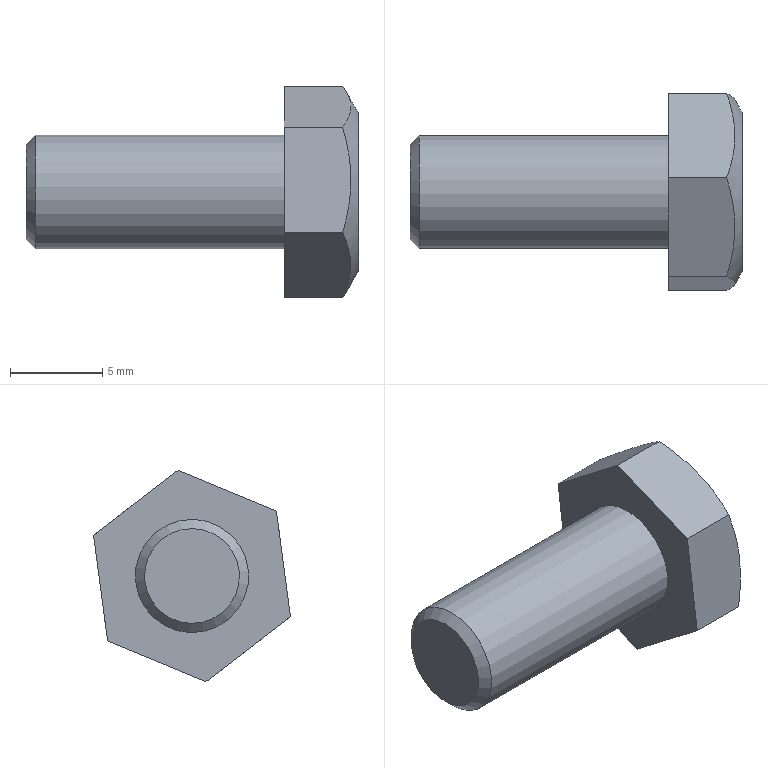Component | NX | BOLT_M6X30 | 1 solid | 12 faces | box 18 x 10.67 x 11.45 mm | volume 751 mm3 | plane 9 | cone 2 | cylinder 1 | commonest cylinder face diameters 6.144 x1
STEP:
#1=CARTESIAN_POINT('',(0.,0.,0.));
#2=DIRECTION('',(0.,0.,1.));
#3=DIRECTION('',(1.,0.,0.));
#4=AXIS2_PLACEMENT_3D('',#1,#2,#3);
#5=CARTESIAN_POINT('',(11.5,2.377,-2.015));
#6=VERTEX_POINT('',#5);
#7=CARTESIAN_POINT('',(11.5,0.,-2.997));
#8=DIRECTION('',(-1.,0.,0.));
#9=DIRECTION('',(0.,0.9242,0.3818));
#10=AXIS2_PLACEMENT_3D('',#7,#8,#9);
#11=CIRCLE('',#10,2.572);
#12=CARTESIAN_POINT('',(11.5,0.,-2.997));
#13=DIRECTION('',(-1.,0.,0.));
#14=DIRECTION('',(0.,0.9242,0.3818));
#15=AXIS2_PLACEMENT_3D('',#12,#13,#14);
#16=PLANE('',#15);
#17=CARTESIAN_POINT('',(0.,0.));
#18=DIRECTION('',(1.,0.));
#19=AXIS2_PLACEMENT_2D('',#17,#18);
#20=CIRCLE('',#19,2.572);
#21=(GEOMETRIC_REPRESENTATION_CONTEXT(2)PARAMETRIC_REPRESENTATION_CONTEXT()REPRESENTATION_CONTEXT('',''));
#22=DEFINITIONAL_REPRESENTATION('',(#20),#21);
#23=PCURVE('',#16,#22);
#24=CARTESIAN_POINT('',(12.,0.,-2.997));
#25=DIRECTION('',(1.,0.,0.));
#26=DIRECTION('',(0.,-0.9242,-0.3818));
#27=AXIS2_PLACEMENT_3D('',#24,#25,#26);
#28=CONICAL_SURFACE('',#27,3.072,0.7854);
#29=CARTESIAN_POINT('',(9.425,-0.5));
#30=DIRECTION('',(-1.,-0.));
#31=VECTOR('',#30,1.);
#32=LINE('',#29,#31);
#33=(GEOMETRIC_REPRESENTATION_CONTEXT(2)PARAMETRIC_REPRESENTATION_CONTEXT()REPRESENTATION_CONTEXT('',''));
#34=DEFINITIONAL_REPRESENTATION('',(#32),#33);
#35=PCURVE('',#28,#34);
#36=SURFACE_CURVE('',#11,(#23,#35),.PCURVE_S1.);
#37=EDGE_CURVE('',#6,#6,#36,.T.);
#38=ORIENTED_EDGE('',*,*,#37,.T.);
#39=EDGE_LOOP('',(#38));
#40=FACE_BOUND('',#39,.T.);
#41=ADVANCED_FACE('',(#40),#16,.T.);
#42=CARTESIAN_POINT('',(12.,2.839,-1.824));
#43=VERTEX_POINT('',#42);
#44=CARTESIAN_POINT('',(12.,-2.839,-4.17));
#45=VERTEX_POINT('',#44);
#46=CARTESIAN_POINT('',(12.,0.,-2.997));
#47=DIRECTION('',(1.,0.,0.));
#48=DIRECTION('',(0.,0.9242,0.3818));
#49=AXIS2_PLACEMENT_3D('',#46,#47,#48);
#50=CIRCLE('',#49,3.072);
#51=CARTESIAN_POINT('',(11.5,0.,-2.997));
#52=DIRECTION('',(1.,0.,0.));
#53=DIRECTION('',(0.,-0.9242,-0.3818));
#54=AXIS2_PLACEMENT_3D('',#51,#52,#53);
#55=CYLINDRICAL_SURFACE('',#54,3.072);
#56=CARTESIAN_POINT('',(3.142,0.5));
#57=DIRECTION('',(1.,0.));
#58=VECTOR('',#57,1.);
#59=LINE('',#56,#58);
#60=(GEOMETRIC_REPRESENTATION_CONTEXT(2)PARAMETRIC_REPRESENTATION_CONTEXT()REPRESENTATION_CONTEXT('',''));
#61=DEFINITIONAL_REPRESENTATION('',(#59),#60);
#62=PCURVE('',#55,#61);
#63=CARTESIAN_POINT('',(3.142,0.));
#64=DIRECTION('',(1.,0.));
#65=VECTOR('',#64,1.);
#66=LINE('',#63,#65);
#67=(GEOMETRIC_REPRESENTATION_CONTEXT(2)PARAMETRIC_REPRESENTATION_CONTEXT()REPRESENTATION_CONTEXT('',''));
#68=DEFINITIONAL_REPRESENTATION('',(#66),#67);
#69=PCURVE('',#28,#68);
#70=SURFACE_CURVE('',#50,(#62,#69),.PCURVE_S1.);
#71=EDGE_CURVE('',#43,#45,#70,.T.);
#72=ORIENTED_EDGE('',*,*,#71,.T.);
#73=CARTESIAN_POINT('',(25.5,-2.839,-4.17));
#74=VERTEX_POINT('',#73);
#75=CARTESIAN_POINT('',(12.,-2.839,-4.17));
#76=CARTESIAN_POINT('',(25.5,-2.839,-4.17));
#77=B_SPLINE_CURVE_WITH_KNOTS('',1,(#75,#76),.UNSPECIFIED.,.F.,.F.,(2,2),(0.5,14.),.PIECEWISE_BEZIER_KNOTS.);
#78=CARTESIAN_POINT('',(6.283,0.));
#79=DIRECTION('',(0.,1.));
#80=VECTOR('',#79,1.);
#81=LINE('',#78,#80);
#82=(GEOMETRIC_REPRESENTATION_CONTEXT(2)PARAMETRIC_REPRESENTATION_CONTEXT()REPRESENTATION_CONTEXT('',''));
#83=DEFINITIONAL_REPRESENTATION('',(#81),#82);
#84=PCURVE('',#55,#83);
#85=CARTESIAN_POINT('',(0.,0.));
#86=DIRECTION('',(0.,1.));
#87=VECTOR('',#86,1.);
#88=LINE('',#85,#87);
#89=(GEOMETRIC_REPRESENTATION_CONTEXT(2)PARAMETRIC_REPRESENTATION_CONTEXT()REPRESENTATION_CONTEXT('',''));
#90=DEFINITIONAL_REPRESENTATION('',(#88),#89);
#91=PCURVE('',#55,#90);
#92=SEAM_CURVE('',#77,(#84,#91),.PCURVE_S1.);
#93=EDGE_CURVE('',#45,#74,#92,.T.);
#94=ORIENTED_EDGE('',*,*,#93,.T.);
#95=CARTESIAN_POINT('',(25.5,0.,-2.997));
#96=DIRECTION('',(-1.,0.,0.));
#97=DIRECTION('',(0.,-0.9242,-0.3818));
#98=AXIS2_PLACEMENT_3D('',#95,#96,#97);
#99=CIRCLE('',#98,3.072);
#100=CARTESIAN_POINT('',(6.283,14.));
#101=DIRECTION('',(-1.,0.));
#102=VECTOR('',#101,1.);
#103=LINE('',#100,#102);
#104=(GEOMETRIC_REPRESENTATION_CONTEXT(2)PARAMETRIC_REPRESENTATION_CONTEXT()REPRESENTATION_CONTEXT('',''));
#105=DEFINITIONAL_REPRESENTATION('',(#103),#104);
#106=PCURVE('',#55,#105);
#107=CARTESIAN_POINT('',(25.5,0.,-2.997));
#108=DIRECTION('',(-1.,0.,0.));
#109=DIRECTION('',(0.,0.9242,0.3818));
#110=AXIS2_PLACEMENT_3D('',#107,#108,#109);
#111=PLANE('',#110);
#112=CARTESIAN_POINT('',(0.,0.));
#113=DIRECTION('',(-1.,0.));
#114=AXIS2_PLACEMENT_2D('',#112,#113);
#115=CIRCLE('',#114,3.072);
#116=(GEOMETRIC_REPRESENTATION_CONTEXT(2)PARAMETRIC_REPRESENTATION_CONTEXT()REPRESENTATION_CONTEXT('',''));
#117=DEFINITIONAL_REPRESENTATION('',(#115),#116);
#118=PCURVE('',#111,#117);
#119=SURFACE_CURVE('',#99,(#106,#118),.PCURVE_S1.);
#120=EDGE_CURVE('',#74,#74,#119,.T.);
#121=ORIENTED_EDGE('',*,*,#120,.T.);
#122=ORIENTED_EDGE('',*,*,#93,.F.);
#123=CARTESIAN_POINT('',(12.,0.,-2.997));
#124=DIRECTION('',(1.,0.,0.));
#125=DIRECTION('',(0.,0.9242,0.3818));
#126=AXIS2_PLACEMENT_3D('',#123,#124,#125);
#127=CIRCLE('',#126,3.072);
#128=CARTESIAN_POINT('',(-3.142,0.5));
#129=DIRECTION('',(1.,0.));
#130=VECTOR('',#129,1.);
#131=LINE('',#128,#130);
#132=(GEOMETRIC_REPRESENTATION_CONTEXT(2)PARAMETRIC_REPRESENTATION_CONTEXT()REPRESENTATION_CONTEXT('',''));
#133=DEFINITIONAL_REPRESENTATION('',(#131),#132);
#134=PCURVE('',#55,#133);
#135=CARTESIAN_POINT('',(3.142,-0.));
#136=DIRECTION('',(1.,0.));
#137=VECTOR('',#136,1.);
#138=LINE('',#135,#137);
#139=(GEOMETRIC_REPRESENTATION_CONTEXT(2)PARAMETRIC_REPRESENTATION_CONTEXT()REPRESENTATION_CONTEXT('',''));
#140=DEFINITIONAL_REPRESENTATION('',(#138),#139);
#141=PCURVE('',#28,#140);
#142=SURFACE_CURVE('',#127,(#134,#141),.PCURVE_S1.);
#143=EDGE_CURVE('',#45,#43,#142,.T.);
#144=ORIENTED_EDGE('',*,*,#143,.T.);
#145=EDGE_LOOP('',(#72,#94,#121,#122,#144));
#146=FACE_BOUND('',#145,.T.);
#147=ADVANCED_FACE('',(#146),#55,.T.);
#148=CARTESIAN_POINT('',(28.667,-5.336,-5.201));
#149=VERTEX_POINT('',#148);
#150=CARTESIAN_POINT('',(28.667,-0.7588,-8.72));
#151=VERTEX_POINT('',#150);
#152=CARTESIAN_POINT('',(28.667,-5.336,-5.201));
#153=CARTESIAN_POINT('',(28.939,-4.589,-5.776));
#154=CARTESIAN_POINT('',(29.113,-3.83,-6.359));
#155=CARTESIAN_POINT('',(29.114,-2.273,-7.556));
#156=CARTESIAN_POINT('',(28.939,-1.507,-8.145));
#157=CARTESIAN_POINT('',(28.667,-0.7588,-8.72));
#158=B_SPLINE_CURVE_WITH_KNOTS('',3,(#152,#153,#154,#155,#156,#157),.UNSPECIFIED.,.F.,.F.,(4,2,4),(0.,0.5,1.),.UNSPECIFIED.);
#159=CARTESIAN_POINT('',(29.5,-0.7588,-8.72));
#160=DIRECTION('',(0.,-0.6095,-0.7928));
#161=DIRECTION('',(0.,0.7928,-0.6095));
#162=AXIS2_PLACEMENT_3D('',#159,#160,#161);
#163=PLANE('',#162);
#164=CARTESIAN_POINT('',(-5.774,-0.8333));
#165=CARTESIAN_POINT('',(-4.831,-0.5612));
#166=CARTESIAN_POINT('',(-3.874,-0.3874));
#167=CARTESIAN_POINT('',(-1.911,-0.3861));
#168=CARTESIAN_POINT('',(-0.9439,-0.5609));
#169=CARTESIAN_POINT('',(0.,-0.8333));
#170=B_SPLINE_CURVE_WITH_KNOTS('',3,(#164,#165,#166,#167,#168,#169),.UNSPECIFIED.,.F.,.F.,(4,2,4),(0.,0.5,1.),.UNSPECIFIED.);
#171=(GEOMETRIC_REPRESENTATION_CONTEXT(2)PARAMETRIC_REPRESENTATION_CONTEXT()REPRESENTATION_CONTEXT('',''));
#172=DEFINITIONAL_REPRESENTATION('',(#170),#171);
#173=PCURVE('',#163,#172);
#174=CARTESIAN_POINT('',(29.5,0.,-2.997));
#175=DIRECTION('',(-1.,0.,0.));
#176=DIRECTION('',(0.,0.9242,0.3818));
#177=AXIS2_PLACEMENT_3D('',#174,#175,#176);
#178=CONICAL_SURFACE('',#177,4.33,1.047);
#179=CARTESIAN_POINT('',(3.142,0.8333));
#180=CARTESIAN_POINT('',(3.129,0.8086));
#181=CARTESIAN_POINT('',(3.102,0.7607));
#182=CARTESIAN_POINT('',(3.061,0.694));
#183=CARTESIAN_POINT('',(3.018,0.6329));
#184=CARTESIAN_POINT('',(2.973,0.5776));
#185=CARTESIAN_POINT('',(2.926,0.5285));
#186=CARTESIAN_POINT('',(2.878,0.4861));
#187=CARTESIAN_POINT('',(2.828,0.4507));
#188=CARTESIAN_POINT('',(2.777,0.4227));
#189=CARTESIAN_POINT('',(2.725,0.4022));
#190=CARTESIAN_POINT('',(2.673,0.3897));
#191=CARTESIAN_POINT('',(2.619,0.3854));
#192=CARTESIAN_POINT('',(2.566,0.3894));
#193=CARTESIAN_POINT('',(2.513,0.4016));
#194=CARTESIAN_POINT('',(2.46,0.4219));
#195=CARTESIAN_POINT('',(2.409,0.4498));
#196=CARTESIAN_POINT('',(2.359,0.4852));
#197=CARTESIAN_POINT('',(2.311,0.5277));
#198=CARTESIAN_POINT('',(2.264,0.5769));
#199=CARTESIAN_POINT('',(2.218,0.6323));
#200=CARTESIAN_POINT('',(2.175,0.6937));
#201=CARTESIAN_POINT('',(2.134,0.7606));
#202=CARTESIAN_POINT('',(2.107,0.8086));
#203=CARTESIAN_POINT('',(2.094,0.8333));
#204=B_SPLINE_CURVE_WITH_KNOTS('',3,(#179,#180,#181,#182,#183,#184,#185,#186,#187,#188,#189,#190,#191,#192,#193,#194,#195,#196,#197,#198,#199,#200,#201,#202,#203),.UNSPECIFIED.,.F.,.F.,(4,1,1,1,1,1,1,1,1,1,1,1,1,1,1,1,1,1,1,1,1,1,4),(0.,0.04545,0.09091,0.1364,0.1818,0.2273,0.2727,0.3182,0.3636,0.4091,0.4545,0.5,0.5455,0.5909,0.6364,0.6818,0.7273,0.7727,0.8182,0.8636,0.9091,0.9545,1.),.QUASI_UNIFORM_KNOTS.);
#205=(GEOMETRIC_REPRESENTATION_CONTEXT(2)PARAMETRIC_REPRESENTATION_CONTEXT()REPRESENTATION_CONTEXT('',''));
#206=DEFINITIONAL_REPRESENTATION('',(#204),#205);
#207=PCURVE('',#178,#206);
#208=SURFACE_CURVE('',#158,(#173,#207),.PCURVE_S1.);
#209=EDGE_CURVE('',#149,#151,#208,.T.);
#210=ORIENTED_EDGE('',*,*,#209,.F.);
#211=CARTESIAN_POINT('',(25.5,-5.336,-5.201));
#212=VERTEX_POINT('',#211);
#213=CARTESIAN_POINT('',(29.5,-5.336,-5.201));
#214=DIRECTION('',(-1.,0.,0.));
#215=VECTOR('',#214,1.);
#216=LINE('',#213,#215);
#217=CARTESIAN_POINT('',(-5.774,0.));
#218=DIRECTION('',(0.,-1.));
#219=VECTOR('',#218,1.);
#220=LINE('',#217,#219);
#221=(GEOMETRIC_REPRESENTATION_CONTEXT(2)PARAMETRIC_REPRESENTATION_CONTEXT()REPRESENTATION_CONTEXT('',''));
#222=DEFINITIONAL_REPRESENTATION('',(#220),#221);
#223=PCURVE('',#163,#222);
#224=CARTESIAN_POINT('',(29.5,-5.336,-5.201));
#225=DIRECTION('',(0.,-0.9913,0.1314));
#226=DIRECTION('',(0.,-0.1314,-0.9913));
#227=AXIS2_PLACEMENT_3D('',#224,#225,#226);
#228=PLANE('',#227);
#229=CARTESIAN_POINT('',(0.,0.));
#230=DIRECTION('',(0.,-1.));
#231=VECTOR('',#230,1.);
#232=LINE('',#229,#231);
#233=(GEOMETRIC_REPRESENTATION_CONTEXT(2)PARAMETRIC_REPRESENTATION_CONTEXT()REPRESENTATION_CONTEXT('',''));
#234=DEFINITIONAL_REPRESENTATION('',(#232),#233);
#235=PCURVE('',#228,#234);
#236=SURFACE_CURVE('',#216,(#223,#235),.PCURVE_S1.);
#237=EDGE_CURVE('',#149,#212,#236,.T.);
#238=ORIENTED_EDGE('',*,*,#237,.T.);
#239=CARTESIAN_POINT('',(25.5,-0.7588,-8.72));
#240=VERTEX_POINT('',#239);
#241=CARTESIAN_POINT('',(25.5,-0.7588,-8.72));
#242=DIRECTION('',(0.,-0.7928,0.6095));
#243=VECTOR('',#242,1.);
#244=LINE('',#241,#243);
#245=CARTESIAN_POINT('',(0.,-4.));
#246=DIRECTION('',(-1.,0.));
#247=VECTOR('',#246,1.);
#248=LINE('',#245,#247);
#249=(GEOMETRIC_REPRESENTATION_CONTEXT(2)PARAMETRIC_REPRESENTATION_CONTEXT()REPRESENTATION_CONTEXT('',''));
#250=DEFINITIONAL_REPRESENTATION('',(#248),#249);
#251=PCURVE('',#163,#250);
#252=CARTESIAN_POINT('',(-2.887,5.));
#253=DIRECTION('',(-0.5,-0.866));
#254=VECTOR('',#253,1.);
#255=LINE('',#252,#254);
#256=(GEOMETRIC_REPRESENTATION_CONTEXT(2)PARAMETRIC_REPRESENTATION_CONTEXT()REPRESENTATION_CONTEXT('',''));
#257=DEFINITIONAL_REPRESENTATION('',(#255),#256);
#258=PCURVE('',#111,#257);
#259=SURFACE_CURVE('',#244,(#251,#258),.PCURVE_S1.);
#260=EDGE_CURVE('',#240,#212,#259,.T.);
#261=ORIENTED_EDGE('',*,*,#260,.F.);
#262=CARTESIAN_POINT('',(29.5,-0.7588,-8.72));
#263=DIRECTION('',(-1.,0.,0.));
#264=VECTOR('',#263,1.);
#265=LINE('',#262,#264);
#266=CARTESIAN_POINT('',(0.,0.));
#267=DIRECTION('',(0.,-1.));
#268=VECTOR('',#267,1.);
#269=LINE('',#266,#268);
#270=(GEOMETRIC_REPRESENTATION_CONTEXT(2)PARAMETRIC_REPRESENTATION_CONTEXT()REPRESENTATION_CONTEXT('',''));
#271=DEFINITIONAL_REPRESENTATION('',(#269),#270);
#272=PCURVE('',#163,#271);
#273=CARTESIAN_POINT('',(29.5,4.577,-6.516));
#274=DIRECTION('',(0.,0.3818,-0.9242));
#275=DIRECTION('',(0.,0.9242,0.3818));
#276=AXIS2_PLACEMENT_3D('',#273,#274,#275);
#277=PLANE('',#276);
#278=CARTESIAN_POINT('',(-5.774,0.));
#279=DIRECTION('',(0.,-1.));
#280=VECTOR('',#279,1.);
#281=LINE('',#278,#280);
#282=(GEOMETRIC_REPRESENTATION_CONTEXT(2)PARAMETRIC_REPRESENTATION_CONTEXT()REPRESENTATION_CONTEXT('',''));
#283=DEFINITIONAL_REPRESENTATION('',(#281),#282);
#284=PCURVE('',#277,#283);
#285=SURFACE_CURVE('',#265,(#272,#284),.PCURVE_S1.);
#286=EDGE_CURVE('',#151,#240,#285,.T.);
#287=ORIENTED_EDGE('',*,*,#286,.F.);
#288=EDGE_LOOP('',(#210,#238,#261,#287));
#289=FACE_BOUND('',#288,.T.);
#290=ADVANCED_FACE('',(#289),#163,.T.);
#291=CARTESIAN_POINT('',(28.667,-4.577,0.522));
#292=VERTEX_POINT('',#291);
#293=CARTESIAN_POINT('',(28.667,-4.577,0.522));
#294=CARTESIAN_POINT('',(28.939,-4.701,-0.4125));
#295=CARTESIAN_POINT('',(29.113,-4.827,-1.361));
#296=CARTESIAN_POINT('',(29.114,-5.085,-3.307));
#297=CARTESIAN_POINT('',(28.939,-5.212,-4.266));
#298=CARTESIAN_POINT('',(28.667,-5.336,-5.201));
#299=B_SPLINE_CURVE_WITH_KNOTS('',3,(#293,#294,#295,#296,#297,#298),.UNSPECIFIED.,.F.,.F.,(4,2,4),(0.,0.5,1.),.UNSPECIFIED.);
#300=CARTESIAN_POINT('',(-5.774,-0.8333));
#301=CARTESIAN_POINT('',(-4.831,-0.5612));
#302=CARTESIAN_POINT('',(-3.874,-0.3874));
#303=CARTESIAN_POINT('',(-1.911,-0.3861));
#304=CARTESIAN_POINT('',(-0.9439,-0.5609));
#305=CARTESIAN_POINT('',(0.,-0.8333));
#306=B_SPLINE_CURVE_WITH_KNOTS('',3,(#300,#301,#302,#303,#304,#305),.UNSPECIFIED.,.F.,.F.,(4,2,4),(0.,0.5,1.),.UNSPECIFIED.);
#307=(GEOMETRIC_REPRESENTATION_CONTEXT(2)PARAMETRIC_REPRESENTATION_CONTEXT()REPRESENTATION_CONTEXT('',''));
#308=DEFINITIONAL_REPRESENTATION('',(#306),#307);
#309=PCURVE('',#228,#308);
#310=CARTESIAN_POINT('',(4.189,0.8333));
#311=CARTESIAN_POINT('',(4.176,0.8086));
#312=CARTESIAN_POINT('',(4.15,0.7607));
#313=CARTESIAN_POINT('',(4.108,0.694));
#314=CARTESIAN_POINT('',(4.065,0.6329));
#315=CARTESIAN_POINT('',(4.02,0.5776));
#316=CARTESIAN_POINT('',(3.974,0.5285));
#317=CARTESIAN_POINT('',(3.925,0.4861));
#318=CARTESIAN_POINT('',(3.876,0.4507));
#319=CARTESIAN_POINT('',(3.825,0.4227));
#320=CARTESIAN_POINT('',(3.773,0.4022));
#321=CARTESIAN_POINT('',(3.72,0.3897));
#322=CARTESIAN_POINT('',(3.666,0.3854));
#323=CARTESIAN_POINT('',(3.613,0.3894));
#324=CARTESIAN_POINT('',(3.56,0.4016));
#325=CARTESIAN_POINT('',(3.507,0.4219));
#326=CARTESIAN_POINT('',(3.456,0.4498));
#327=CARTESIAN_POINT('',(3.406,0.4852));
#328=CARTESIAN_POINT('',(3.358,0.5277));
#329=CARTESIAN_POINT('',(3.311,0.5769));
#330=CARTESIAN_POINT('',(3.266,0.6323));
#331=CARTESIAN_POINT('',(3.222,0.6937));
#332=CARTESIAN_POINT('',(3.181,0.7606));
#333=CARTESIAN_POINT('',(3.154,0.8086));
#334=CARTESIAN_POINT('',(3.142,0.8333));
#335=B_SPLINE_CURVE_WITH_KNOTS('',3,(#310,#311,#312,#313,#314,#315,#316,#317,#318,#319,#320,#321,#322,#323,#324,#325,#326,#327,#328,#329,#330,#331,#332,#333,#334),.UNSPECIFIED.,.F.,.F.,(4,1,1,1,1,1,1,1,1,1,1,1,1,1,1,1,1,1,1,1,1,1,4),(0.,0.04545,0.09091,0.1364,0.1818,0.2273,0.2727,0.3182,0.3636,0.4091,0.4545,0.5,0.5455,0.5909,0.6364,0.6818,0.7273,0.7727,0.8182,0.8636,0.9091,0.9545,1.),.QUASI_UNIFORM_KNOTS.);
#336=(GEOMETRIC_REPRESENTATION_CONTEXT(2)PARAMETRIC_REPRESENTATION_CONTEXT()REPRESENTATION_CONTEXT('',''));
#337=DEFINITIONAL_REPRESENTATION('',(#335),#336);
#338=PCURVE('',#178,#337);
#339=SURFACE_CURVE('',#299,(#309,#338),.PCURVE_S1.);
#340=EDGE_CURVE('',#292,#149,#339,.T.);
#341=ORIENTED_EDGE('',*,*,#340,.F.);
#342=CARTESIAN_POINT('',(25.5,-4.577,0.522));
#343=VERTEX_POINT('',#342);
#344=CARTESIAN_POINT('',(29.5,-4.577,0.522));
#345=DIRECTION('',(-1.,0.,0.));
#346=VECTOR('',#345,1.);
#347=LINE('',#344,#346);
#348=CARTESIAN_POINT('',(-5.774,0.));
#349=DIRECTION('',(0.,-1.));
#350=VECTOR('',#349,1.);
#351=LINE('',#348,#350);
#352=(GEOMETRIC_REPRESENTATION_CONTEXT(2)PARAMETRIC_REPRESENTATION_CONTEXT()REPRESENTATION_CONTEXT('',''));
#353=DEFINITIONAL_REPRESENTATION('',(#351),#352);
#354=PCURVE('',#228,#353);
#355=CARTESIAN_POINT('',(29.5,-4.577,0.522));
#356=DIRECTION('',(0.,-0.3818,0.9242));
#357=DIRECTION('',(0.,-0.9242,-0.3818));
#358=AXIS2_PLACEMENT_3D('',#355,#356,#357);
#359=PLANE('',#358);
#360=CARTESIAN_POINT('',(0.,0.));
#361=DIRECTION('',(0.,-1.));
#362=VECTOR('',#361,1.);
#363=LINE('',#360,#362);
#364=(GEOMETRIC_REPRESENTATION_CONTEXT(2)PARAMETRIC_REPRESENTATION_CONTEXT()REPRESENTATION_CONTEXT('',''));
#365=DEFINITIONAL_REPRESENTATION('',(#363),#364);
#366=PCURVE('',#359,#365);
#367=SURFACE_CURVE('',#347,(#354,#366),.PCURVE_S1.);
#368=EDGE_CURVE('',#292,#343,#367,.T.);
#369=ORIENTED_EDGE('',*,*,#368,.T.);
#370=CARTESIAN_POINT('',(25.5,-5.336,-5.201));
#371=DIRECTION('',(0.,0.1314,0.9913));
#372=VECTOR('',#371,1.);
#373=LINE('',#370,#372);
#374=CARTESIAN_POINT('',(0.,-4.));
#375=DIRECTION('',(-1.,0.));
#376=VECTOR('',#375,1.);
#377=LINE('',#374,#376);
#378=(GEOMETRIC_REPRESENTATION_CONTEXT(2)PARAMETRIC_REPRESENTATION_CONTEXT()REPRESENTATION_CONTEXT('',''));
#379=DEFINITIONAL_REPRESENTATION('',(#377),#378);
#380=PCURVE('',#228,#379);
#381=CARTESIAN_POINT('',(-5.774,-0.));
#382=DIRECTION('',(0.5,-0.866));
#383=VECTOR('',#382,1.);
#384=LINE('',#381,#383);
#385=(GEOMETRIC_REPRESENTATION_CONTEXT(2)PARAMETRIC_REPRESENTATION_CONTEXT()REPRESENTATION_CONTEXT('',''));
#386=DEFINITIONAL_REPRESENTATION('',(#384),#385);
#387=PCURVE('',#111,#386);
#388=SURFACE_CURVE('',#373,(#380,#387),.PCURVE_S1.);
#389=EDGE_CURVE('',#212,#343,#388,.T.);
#390=ORIENTED_EDGE('',*,*,#389,.F.);
#391=ORIENTED_EDGE('',*,*,#237,.F.);
#392=EDGE_LOOP('',(#341,#369,#390,#391));
#393=FACE_BOUND('',#392,.T.);
#394=ADVANCED_FACE('',(#393),#228,.T.);
#395=CARTESIAN_POINT('',(28.667,0.7588,2.727));
#396=VERTEX_POINT('',#395);
#397=CARTESIAN_POINT('',(28.667,0.7588,2.727));
#398=CARTESIAN_POINT('',(28.938,-0.109,2.368));
#399=CARTESIAN_POINT('',(29.113,-1.008,1.997));
#400=CARTESIAN_POINT('',(29.113,-2.812,1.251));
#401=CARTESIAN_POINT('',(28.936,-3.715,0.8783));
#402=CARTESIAN_POINT('',(28.667,-4.577,0.522));
#403=B_SPLINE_CURVE_WITH_KNOTS('',3,(#397,#398,#399,#400,#401,#402),.UNSPECIFIED.,.F.,.F.,(4,2,4),(0.,0.5,1.),.UNSPECIFIED.);
#404=CARTESIAN_POINT('',(-5.774,-0.8333));
#405=CARTESIAN_POINT('',(-4.835,-0.5623));
#406=CARTESIAN_POINT('',(-3.862,-0.3867));
#407=CARTESIAN_POINT('',(-1.91,-0.3868));
#408=CARTESIAN_POINT('',(-0.9332,-0.5639));
#409=CARTESIAN_POINT('',(0.,-0.8333));
#410=B_SPLINE_CURVE_WITH_KNOTS('',3,(#404,#405,#406,#407,#408,#409),.UNSPECIFIED.,.F.,.F.,(4,2,4),(0.,0.5,1.),.UNSPECIFIED.);
#411=(GEOMETRIC_REPRESENTATION_CONTEXT(2)PARAMETRIC_REPRESENTATION_CONTEXT()REPRESENTATION_CONTEXT('',''));
#412=DEFINITIONAL_REPRESENTATION('',(#410),#411);
#413=PCURVE('',#359,#412);
#414=CARTESIAN_POINT('',(5.236,0.8333));
#415=CARTESIAN_POINT('',(5.223,0.8087));
#416=CARTESIAN_POINT('',(5.197,0.7609));
#417=CARTESIAN_POINT('',(5.156,0.6942));
#418=CARTESIAN_POINT('',(5.112,0.6329));
#419=CARTESIAN_POINT('',(5.067,0.5774));
#420=CARTESIAN_POINT('',(5.02,0.5282));
#421=CARTESIAN_POINT('',(4.972,0.4856));
#422=CARTESIAN_POINT('',(4.922,0.4502));
#423=CARTESIAN_POINT('',(4.87,0.4221));
#424=CARTESIAN_POINT('',(4.818,0.4018));
#425=CARTESIAN_POINT('',(4.765,0.3895));
#426=CARTESIAN_POINT('',(4.712,0.3854));
#427=CARTESIAN_POINT('',(4.659,0.3896));
#428=CARTESIAN_POINT('',(4.606,0.4019));
#429=CARTESIAN_POINT('',(4.554,0.4224));
#430=CARTESIAN_POINT('',(4.503,0.4505));
#431=CARTESIAN_POINT('',(4.453,0.4861));
#432=CARTESIAN_POINT('',(4.404,0.5287));
#433=CARTESIAN_POINT('',(4.357,0.578));
#434=CARTESIAN_POINT('',(4.312,0.6335));
#435=CARTESIAN_POINT('',(4.269,0.6948));
#436=CARTESIAN_POINT('',(4.228,0.7613));
#437=CARTESIAN_POINT('',(4.202,0.8088));
#438=CARTESIAN_POINT('',(4.189,0.8333));
#439=B_SPLINE_CURVE_WITH_KNOTS('',3,(#414,#415,#416,#417,#418,#419,#420,#421,#422,#423,#424,#425,#426,#427,#428,#429,#430,#431,#432,#433,#434,#435,#436,#437,#438),.UNSPECIFIED.,.F.,.F.,(4,1,1,1,1,1,1,1,1,1,1,1,1,1,1,1,1,1,1,1,1,1,4),(0.,0.04545,0.09091,0.1364,0.1818,0.2273,0.2727,0.3182,0.3636,0.4091,0.4545,0.5,0.5455,0.5909,0.6364,0.6818,0.7273,0.7727,0.8182,0.8636,0.9091,0.9545,1.),.QUASI_UNIFORM_KNOTS.);
#440=(GEOMETRIC_REPRESENTATION_CONTEXT(2)PARAMETRIC_REPRESENTATION_CONTEXT()REPRESENTATION_CONTEXT('',''));
#441=DEFINITIONAL_REPRESENTATION('',(#439),#440);
#442=PCURVE('',#178,#441);
#443=SURFACE_CURVE('',#403,(#413,#442),.PCURVE_S1.);
#444=EDGE_CURVE('',#396,#292,#443,.T.);
#445=ORIENTED_EDGE('',*,*,#444,.F.);
#446=CARTESIAN_POINT('',(25.5,0.7588,2.727));
#447=VERTEX_POINT('',#446);
#448=CARTESIAN_POINT('',(29.5,0.7588,2.727));
#449=DIRECTION('',(-1.,0.,0.));
#450=VECTOR('',#449,1.);
#451=LINE('',#448,#450);
#452=CARTESIAN_POINT('',(-5.774,0.));
#453=DIRECTION('',(0.,-1.));
#454=VECTOR('',#453,1.);
#455=LINE('',#452,#454);
#456=(GEOMETRIC_REPRESENTATION_CONTEXT(2)PARAMETRIC_REPRESENTATION_CONTEXT()REPRESENTATION_CONTEXT('',''));
#457=DEFINITIONAL_REPRESENTATION('',(#455),#456);
#458=PCURVE('',#359,#457);
#459=CARTESIAN_POINT('',(29.5,0.7588,2.727));
#460=DIRECTION('',(0.,0.6095,0.7928));
#461=DIRECTION('',(0.,-0.7928,0.6095));
#462=AXIS2_PLACEMENT_3D('',#459,#460,#461);
#463=PLANE('',#462);
#464=CARTESIAN_POINT('',(0.,0.));
#465=DIRECTION('',(0.,-1.));
#466=VECTOR('',#465,1.);
#467=LINE('',#464,#466);
#468=(GEOMETRIC_REPRESENTATION_CONTEXT(2)PARAMETRIC_REPRESENTATION_CONTEXT()REPRESENTATION_CONTEXT('',''));
#469=DEFINITIONAL_REPRESENTATION('',(#467),#468);
#470=PCURVE('',#463,#469);
#471=SURFACE_CURVE('',#451,(#458,#470),.PCURVE_S1.);
#472=EDGE_CURVE('',#396,#447,#471,.T.);
#473=ORIENTED_EDGE('',*,*,#472,.T.);
#474=CARTESIAN_POINT('',(25.5,-4.577,0.522));
#475=DIRECTION('',(0.,0.9242,0.3818));
#476=VECTOR('',#475,1.);
#477=LINE('',#474,#476);
#478=CARTESIAN_POINT('',(0.,-4.));
#479=DIRECTION('',(-1.,0.));
#480=VECTOR('',#479,1.);
#481=LINE('',#478,#480);
#482=(GEOMETRIC_REPRESENTATION_CONTEXT(2)PARAMETRIC_REPRESENTATION_CONTEXT()REPRESENTATION_CONTEXT('',''));
#483=DEFINITIONAL_REPRESENTATION('',(#481),#482);
#484=PCURVE('',#359,#483);
#485=CARTESIAN_POINT('',(-2.887,-5.));
#486=DIRECTION('',(1.,0.));
#487=VECTOR('',#486,1.);
#488=LINE('',#485,#487);
#489=(GEOMETRIC_REPRESENTATION_CONTEXT(2)PARAMETRIC_REPRESENTATION_CONTEXT()REPRESENTATION_CONTEXT('',''));
#490=DEFINITIONAL_REPRESENTATION('',(#488),#489);
#491=PCURVE('',#111,#490);
#492=SURFACE_CURVE('',#477,(#484,#491),.PCURVE_S1.);
#493=EDGE_CURVE('',#343,#447,#492,.T.);
#494=ORIENTED_EDGE('',*,*,#493,.F.);
#495=ORIENTED_EDGE('',*,*,#368,.F.);
#496=EDGE_LOOP('',(#445,#473,#494,#495));
#497=FACE_BOUND('',#496,.T.);
#498=ADVANCED_FACE('',(#497),#359,.T.);
#499=CARTESIAN_POINT('',(28.667,5.336,-0.7922));
#500=VERTEX_POINT('',#499);
#501=CARTESIAN_POINT('',(28.667,5.336,-0.7922));
#502=CARTESIAN_POINT('',(28.939,4.589,-0.2177));
#503=CARTESIAN_POINT('',(29.113,3.83,0.3655));
#504=CARTESIAN_POINT('',(29.114,2.273,1.562));
#505=CARTESIAN_POINT('',(28.939,1.507,2.151));
#506=CARTESIAN_POINT('',(28.667,0.7588,2.727));
#507=B_SPLINE_CURVE_WITH_KNOTS('',3,(#501,#502,#503,#504,#505,#506),.UNSPECIFIED.,.F.,.F.,(4,2,4),(0.,0.5,1.),.UNSPECIFIED.);
#508=CARTESIAN_POINT('',(-5.774,-0.8333));
#509=CARTESIAN_POINT('',(-4.831,-0.5612));
#510=CARTESIAN_POINT('',(-3.874,-0.3874));
#511=CARTESIAN_POINT('',(-1.911,-0.3861));
#512=CARTESIAN_POINT('',(-0.9439,-0.5609));
#513=CARTESIAN_POINT('',(0.,-0.8333));
#514=B_SPLINE_CURVE_WITH_KNOTS('',3,(#508,#509,#510,#511,#512,#513),.UNSPECIFIED.,.F.,.F.,(4,2,4),(0.,0.5,1.),.UNSPECIFIED.);
#515=(GEOMETRIC_REPRESENTATION_CONTEXT(2)PARAMETRIC_REPRESENTATION_CONTEXT()REPRESENTATION_CONTEXT('',''));
#516=DEFINITIONAL_REPRESENTATION('',(#514),#515);
#517=PCURVE('',#463,#516);
#518=CARTESIAN_POINT('',(6.283,0.8333));
#519=CARTESIAN_POINT('',(6.27,0.8086));
#520=CARTESIAN_POINT('',(6.244,0.7607));
#521=CARTESIAN_POINT('',(6.203,0.694));
#522=CARTESIAN_POINT('',(6.16,0.6329));
#523=CARTESIAN_POINT('',(6.115,0.5776));
#524=CARTESIAN_POINT('',(6.068,0.5285));
#525=CARTESIAN_POINT('',(6.02,0.4861));
#526=CARTESIAN_POINT('',(5.97,0.4507));
#527=CARTESIAN_POINT('',(5.919,0.4227));
#528=CARTESIAN_POINT('',(5.867,0.4022));
#529=CARTESIAN_POINT('',(5.814,0.3897));
#530=CARTESIAN_POINT('',(5.761,0.3854));
#531=CARTESIAN_POINT('',(5.707,0.3894));
#532=CARTESIAN_POINT('',(5.654,0.4016));
#533=CARTESIAN_POINT('',(5.602,0.4219));
#534=CARTESIAN_POINT('',(5.551,0.4498));
#535=CARTESIAN_POINT('',(5.501,0.4852));
#536=CARTESIAN_POINT('',(5.452,0.5277));
#537=CARTESIAN_POINT('',(5.405,0.5769));
#538=CARTESIAN_POINT('',(5.36,0.6323));
#539=CARTESIAN_POINT('',(5.317,0.6937));
#540=CARTESIAN_POINT('',(5.275,0.7606));
#541=CARTESIAN_POINT('',(5.249,0.8086));
#542=CARTESIAN_POINT('',(5.236,0.8333));
#543=B_SPLINE_CURVE_WITH_KNOTS('',3,(#518,#519,#520,#521,#522,#523,#524,#525,#526,#527,#528,#529,#530,#531,#532,#533,#534,#535,#536,#537,#538,#539,#540,#541,#542),.UNSPECIFIED.,.F.,.F.,(4,1,1,1,1,1,1,1,1,1,1,1,1,1,1,1,1,1,1,1,1,1,4),(0.,0.04545,0.09091,0.1364,0.1818,0.2273,0.2727,0.3182,0.3636,0.4091,0.4545,0.5,0.5455,0.5909,0.6364,0.6818,0.7273,0.7727,0.8182,0.8636,0.9091,0.9545,1.),.QUASI_UNIFORM_KNOTS.);
#544=(GEOMETRIC_REPRESENTATION_CONTEXT(2)PARAMETRIC_REPRESENTATION_CONTEXT()REPRESENTATION_CONTEXT('',''));
#545=DEFINITIONAL_REPRESENTATION('',(#543),#544);
#546=PCURVE('',#178,#545);
#547=SURFACE_CURVE('',#507,(#517,#546),.PCURVE_S1.);
#548=EDGE_CURVE('',#500,#396,#547,.T.);
#549=ORIENTED_EDGE('',*,*,#548,.F.);
#550=CARTESIAN_POINT('',(25.5,5.336,-0.7922));
#551=VERTEX_POINT('',#550);
#552=CARTESIAN_POINT('',(29.5,5.336,-0.7922));
#553=DIRECTION('',(-1.,0.,0.));
#554=VECTOR('',#553,1.);
#555=LINE('',#552,#554);
#556=CARTESIAN_POINT('',(-5.774,0.));
#557=DIRECTION('',(0.,-1.));
#558=VECTOR('',#557,1.);
#559=LINE('',#556,#558);
#560=(GEOMETRIC_REPRESENTATION_CONTEXT(2)PARAMETRIC_REPRESENTATION_CONTEXT()REPRESENTATION_CONTEXT('',''));
#561=DEFINITIONAL_REPRESENTATION('',(#559),#560);
#562=PCURVE('',#463,#561);
#563=CARTESIAN_POINT('',(29.5,5.336,-0.7922));
#564=DIRECTION('',(0.,0.9913,-0.1314));
#565=DIRECTION('',(0.,0.1314,0.9913));
#566=AXIS2_PLACEMENT_3D('',#563,#564,#565);
#567=PLANE('',#566);
#568=CARTESIAN_POINT('',(0.,0.));
#569=DIRECTION('',(0.,-1.));
#570=VECTOR('',#569,1.);
#571=LINE('',#568,#570);
#572=(GEOMETRIC_REPRESENTATION_CONTEXT(2)PARAMETRIC_REPRESENTATION_CONTEXT()REPRESENTATION_CONTEXT('',''));
#573=DEFINITIONAL_REPRESENTATION('',(#571),#572);
#574=PCURVE('',#567,#573);
#575=SURFACE_CURVE('',#555,(#562,#574),.PCURVE_S1.);
#576=EDGE_CURVE('',#500,#551,#575,.T.);
#577=ORIENTED_EDGE('',*,*,#576,.T.);
#578=CARTESIAN_POINT('',(25.5,0.7588,2.727));
#579=DIRECTION('',(0.,0.7928,-0.6095));
#580=VECTOR('',#579,1.);
#581=LINE('',#578,#580);
#582=CARTESIAN_POINT('',(0.,-4.));
#583=DIRECTION('',(-1.,0.));
#584=VECTOR('',#583,1.);
#585=LINE('',#582,#584);
#586=(GEOMETRIC_REPRESENTATION_CONTEXT(2)PARAMETRIC_REPRESENTATION_CONTEXT()REPRESENTATION_CONTEXT('',''));
#587=DEFINITIONAL_REPRESENTATION('',(#585),#586);
#588=PCURVE('',#463,#587);
#589=CARTESIAN_POINT('',(2.887,-5.));
#590=DIRECTION('',(0.5,0.866));
#591=VECTOR('',#590,1.);
#592=LINE('',#589,#591);
#593=(GEOMETRIC_REPRESENTATION_CONTEXT(2)PARAMETRIC_REPRESENTATION_CONTEXT()REPRESENTATION_CONTEXT('',''));
#594=DEFINITIONAL_REPRESENTATION('',(#592),#593);
#595=PCURVE('',#111,#594);
#596=SURFACE_CURVE('',#581,(#588,#595),.PCURVE_S1.);
#597=EDGE_CURVE('',#447,#551,#596,.T.);
#598=ORIENTED_EDGE('',*,*,#597,.F.);
#599=ORIENTED_EDGE('',*,*,#472,.F.);
#600=EDGE_LOOP('',(#549,#577,#598,#599));
#601=FACE_BOUND('',#600,.T.);
#602=ADVANCED_FACE('',(#601),#463,.T.);
#603=CARTESIAN_POINT('',(28.667,4.577,-6.516));
#604=VERTEX_POINT('',#603);
#605=CARTESIAN_POINT('',(28.667,4.577,-6.516));
#606=CARTESIAN_POINT('',(28.939,4.701,-5.581));
#607=CARTESIAN_POINT('',(29.113,4.827,-4.633));
#608=CARTESIAN_POINT('',(29.114,5.085,-2.686));
#609=CARTESIAN_POINT('',(28.939,5.212,-1.728));
#610=CARTESIAN_POINT('',(28.667,5.336,-0.7922));
#611=B_SPLINE_CURVE_WITH_KNOTS('',3,(#605,#606,#607,#608,#609,#610),.UNSPECIFIED.,.F.,.F.,(4,2,4),(0.,0.5,1.),.UNSPECIFIED.);
#612=CARTESIAN_POINT('',(-5.774,-0.8333));
#613=CARTESIAN_POINT('',(-4.831,-0.5612));
#614=CARTESIAN_POINT('',(-3.874,-0.3874));
#615=CARTESIAN_POINT('',(-1.911,-0.3861));
#616=CARTESIAN_POINT('',(-0.9439,-0.5609));
#617=CARTESIAN_POINT('',(0.,-0.8333));
#618=B_SPLINE_CURVE_WITH_KNOTS('',3,(#612,#613,#614,#615,#616,#617),.UNSPECIFIED.,.F.,.F.,(4,2,4),(0.,0.5,1.),.UNSPECIFIED.);
#619=(GEOMETRIC_REPRESENTATION_CONTEXT(2)PARAMETRIC_REPRESENTATION_CONTEXT()REPRESENTATION_CONTEXT('',''));
#620=DEFINITIONAL_REPRESENTATION('',(#618),#619);
#621=PCURVE('',#567,#620);
#622=CARTESIAN_POINT('',(1.047,0.8333));
#623=CARTESIAN_POINT('',(1.034,0.8086));
#624=CARTESIAN_POINT('',(1.008,0.7607));
#625=CARTESIAN_POINT('',(0.9667,0.694));
#626=CARTESIAN_POINT('',(0.9236,0.6329));
#627=CARTESIAN_POINT('',(0.8787,0.5776));
#628=CARTESIAN_POINT('',(0.832,0.5285));
#629=CARTESIAN_POINT('',(0.7838,0.4861));
#630=CARTESIAN_POINT('',(0.7341,0.4507));
#631=CARTESIAN_POINT('',(0.6831,0.4227));
#632=CARTESIAN_POINT('',(0.631,0.4022));
#633=CARTESIAN_POINT('',(0.5782,0.3897));
#634=CARTESIAN_POINT('',(0.5247,0.3854));
#635=CARTESIAN_POINT('',(0.4712,0.3894));
#636=CARTESIAN_POINT('',(0.4182,0.4016));
#637=CARTESIAN_POINT('',(0.3659,0.4219));
#638=CARTESIAN_POINT('',(0.3147,0.4498));
#639=CARTESIAN_POINT('',(0.2647,0.4852));
#640=CARTESIAN_POINT('',(0.2161,0.5277));
#641=CARTESIAN_POINT('',(0.1692,0.5769));
#642=CARTESIAN_POINT('',(0.124,0.6323));
#643=CARTESIAN_POINT('',(0.0807,0.6937));
#644=CARTESIAN_POINT('',(0.03925,0.7606));
#645=CARTESIAN_POINT('',(0.01287,0.8086));
#646=CARTESIAN_POINT('',(0.,0.8333));
#647=B_SPLINE_CURVE_WITH_KNOTS('',3,(#622,#623,#624,#625,#626,#627,#628,#629,#630,#631,#632,#633,#634,#635,#636,#637,#638,#639,#640,#641,#642,#643,#644,#645,#646),.UNSPECIFIED.,.F.,.F.,(4,1,1,1,1,1,1,1,1,1,1,1,1,1,1,1,1,1,1,1,1,1,4),(0.,0.04545,0.09091,0.1364,0.1818,0.2273,0.2727,0.3182,0.3636,0.4091,0.4545,0.5,0.5455,0.5909,0.6364,0.6818,0.7273,0.7727,0.8182,0.8636,0.9091,0.9545,1.),.QUASI_UNIFORM_KNOTS.);
#648=(GEOMETRIC_REPRESENTATION_CONTEXT(2)PARAMETRIC_REPRESENTATION_CONTEXT()REPRESENTATION_CONTEXT('',''));
#649=DEFINITIONAL_REPRESENTATION('',(#647),#648);
#650=PCURVE('',#178,#649);
#651=SURFACE_CURVE('',#611,(#621,#650),.PCURVE_S1.);
#652=EDGE_CURVE('',#604,#500,#651,.T.);
#653=ORIENTED_EDGE('',*,*,#652,.F.);
#654=CARTESIAN_POINT('',(25.5,4.577,-6.516));
#655=VERTEX_POINT('',#654);
#656=CARTESIAN_POINT('',(29.5,4.577,-6.516));
#657=DIRECTION('',(-1.,0.,0.));
#658=VECTOR('',#657,1.);
#659=LINE('',#656,#658);
#660=CARTESIAN_POINT('',(-5.774,0.));
#661=DIRECTION('',(0.,-1.));
#662=VECTOR('',#661,1.);
#663=LINE('',#660,#662);
#664=(GEOMETRIC_REPRESENTATION_CONTEXT(2)PARAMETRIC_REPRESENTATION_CONTEXT()REPRESENTATION_CONTEXT('',''));
#665=DEFINITIONAL_REPRESENTATION('',(#663),#664);
#666=PCURVE('',#567,#665);
#667=CARTESIAN_POINT('',(0.,0.));
#668=DIRECTION('',(0.,-1.));
#669=VECTOR('',#668,1.);
#670=LINE('',#667,#669);
#671=(GEOMETRIC_REPRESENTATION_CONTEXT(2)PARAMETRIC_REPRESENTATION_CONTEXT()REPRESENTATION_CONTEXT('',''));
#672=DEFINITIONAL_REPRESENTATION('',(#670),#671);
#673=PCURVE('',#277,#672);
#674=SURFACE_CURVE('',#659,(#666,#673),.PCURVE_S1.);
#675=EDGE_CURVE('',#604,#655,#674,.T.);
#676=ORIENTED_EDGE('',*,*,#675,.T.);
#677=CARTESIAN_POINT('',(25.5,5.336,-0.7922));
#678=DIRECTION('',(0.,-0.1314,-0.9913));
#679=VECTOR('',#678,1.);
#680=LINE('',#677,#679);
#681=CARTESIAN_POINT('',(0.,-4.));
#682=DIRECTION('',(-1.,0.));
#683=VECTOR('',#682,1.);
#684=LINE('',#681,#683);
#685=(GEOMETRIC_REPRESENTATION_CONTEXT(2)PARAMETRIC_REPRESENTATION_CONTEXT()REPRESENTATION_CONTEXT('',''));
#686=DEFINITIONAL_REPRESENTATION('',(#684),#685);
#687=PCURVE('',#567,#686);
#688=CARTESIAN_POINT('',(5.774,0.));
#689=DIRECTION('',(-0.5,0.866));
#690=VECTOR('',#689,1.);
#691=LINE('',#688,#690);
#692=(GEOMETRIC_REPRESENTATION_CONTEXT(2)PARAMETRIC_REPRESENTATION_CONTEXT()REPRESENTATION_CONTEXT('',''));
#693=DEFINITIONAL_REPRESENTATION('',(#691),#692);
#694=PCURVE('',#111,#693);
#695=SURFACE_CURVE('',#680,(#687,#694),.PCURVE_S1.);
#696=EDGE_CURVE('',#551,#655,#695,.T.);
#697=ORIENTED_EDGE('',*,*,#696,.F.);
#698=ORIENTED_EDGE('',*,*,#576,.F.);
#699=EDGE_LOOP('',(#653,#676,#697,#698));
#700=FACE_BOUND('',#699,.T.);
#701=ADVANCED_FACE('',(#700),#567,.T.);
#702=CARTESIAN_POINT('',(28.667,-0.7588,-8.72));
#703=CARTESIAN_POINT('',(28.936,0.1038,-8.364));
#704=CARTESIAN_POINT('',(29.113,1.007,-7.991));
#705=CARTESIAN_POINT('',(29.113,2.81,-7.246));
#706=CARTESIAN_POINT('',(28.938,3.709,-6.874));
#707=CARTESIAN_POINT('',(28.667,4.577,-6.516));
#708=B_SPLINE_CURVE_WITH_KNOTS('',3,(#702,#703,#704,#705,#706,#707),.UNSPECIFIED.,.F.,.F.,(4,2,4),(0.,0.5,1.),.UNSPECIFIED.);
#709=CARTESIAN_POINT('',(-5.774,-0.8333));
#710=CARTESIAN_POINT('',(-4.84,-0.5639));
#711=CARTESIAN_POINT('',(-3.863,-0.3868));
#712=CARTESIAN_POINT('',(-1.912,-0.3867));
#713=CARTESIAN_POINT('',(-0.9389,-0.5623));
#714=CARTESIAN_POINT('',(0.,-0.8333));
#715=B_SPLINE_CURVE_WITH_KNOTS('',3,(#709,#710,#711,#712,#713,#714),.UNSPECIFIED.,.F.,.F.,(4,2,4),(0.,0.5,1.),.UNSPECIFIED.);
#716=(GEOMETRIC_REPRESENTATION_CONTEXT(2)PARAMETRIC_REPRESENTATION_CONTEXT()REPRESENTATION_CONTEXT('',''));
#717=DEFINITIONAL_REPRESENTATION('',(#715),#716);
#718=PCURVE('',#277,#717);
#719=CARTESIAN_POINT('',(2.094,0.8333));
#720=CARTESIAN_POINT('',(2.082,0.8088));
#721=CARTESIAN_POINT('',(2.056,0.7613));
#722=CARTESIAN_POINT('',(2.014,0.6948));
#723=CARTESIAN_POINT('',(1.971,0.6335));
#724=CARTESIAN_POINT('',(1.926,0.578));
#725=CARTESIAN_POINT('',(1.879,0.5287));
#726=CARTESIAN_POINT('',(1.831,0.4861));
#727=CARTESIAN_POINT('',(1.781,0.4505));
#728=CARTESIAN_POINT('',(1.729,0.4224));
#729=CARTESIAN_POINT('',(1.677,0.4019));
#730=CARTESIAN_POINT('',(1.624,0.3896));
#731=CARTESIAN_POINT('',(1.571,0.3854));
#732=CARTESIAN_POINT('',(1.518,0.3895));
#733=CARTESIAN_POINT('',(1.465,0.4018));
#734=CARTESIAN_POINT('',(1.413,0.4221));
#735=CARTESIAN_POINT('',(1.362,0.4502));
#736=CARTESIAN_POINT('',(1.312,0.4856));
#737=CARTESIAN_POINT('',(1.263,0.5282));
#738=CARTESIAN_POINT('',(1.216,0.5774));
#739=CARTESIAN_POINT('',(1.171,0.6329));
#740=CARTESIAN_POINT('',(1.128,0.6942));
#741=CARTESIAN_POINT('',(1.086,0.7609));
#742=CARTESIAN_POINT('',(1.06,0.8087));
#743=CARTESIAN_POINT('',(1.047,0.8333));
#744=B_SPLINE_CURVE_WITH_KNOTS('',3,(#719,#720,#721,#722,#723,#724,#725,#726,#727,#728,#729,#730,#731,#732,#733,#734,#735,#736,#737,#738,#739,#740,#741,#742,#743),.UNSPECIFIED.,.F.,.F.,(4,1,1,1,1,1,1,1,1,1,1,1,1,1,1,1,1,1,1,1,1,1,4),(0.,0.04545,0.09091,0.1364,0.1818,0.2273,0.2727,0.3182,0.3636,0.4091,0.4545,0.5,0.5455,0.5909,0.6364,0.6818,0.7273,0.7727,0.8182,0.8636,0.9091,0.9545,1.),.QUASI_UNIFORM_KNOTS.);
#745=(GEOMETRIC_REPRESENTATION_CONTEXT(2)PARAMETRIC_REPRESENTATION_CONTEXT()REPRESENTATION_CONTEXT('',''));
#746=DEFINITIONAL_REPRESENTATION('',(#744),#745);
#747=PCURVE('',#178,#746);
#748=SURFACE_CURVE('',#708,(#718,#747),.PCURVE_S1.);
#749=EDGE_CURVE('',#151,#604,#748,.T.);
#750=ORIENTED_EDGE('',*,*,#749,.F.);
#751=ORIENTED_EDGE('',*,*,#286,.T.);
#752=CARTESIAN_POINT('',(25.5,4.577,-6.516));
#753=DIRECTION('',(0.,-0.9242,-0.3818));
#754=VECTOR('',#753,1.);
#755=LINE('',#752,#754);
#756=CARTESIAN_POINT('',(0.,-4.));
#757=DIRECTION('',(-1.,0.));
#758=VECTOR('',#757,1.);
#759=LINE('',#756,#758);
#760=(GEOMETRIC_REPRESENTATION_CONTEXT(2)PARAMETRIC_REPRESENTATION_CONTEXT()REPRESENTATION_CONTEXT('',''));
#761=DEFINITIONAL_REPRESENTATION('',(#759),#760);
#762=PCURVE('',#277,#761);
#763=CARTESIAN_POINT('',(2.887,5.));
#764=DIRECTION('',(-1.,-0.));
#765=VECTOR('',#764,1.);
#766=LINE('',#763,#765);
#767=(GEOMETRIC_REPRESENTATION_CONTEXT(2)PARAMETRIC_REPRESENTATION_CONTEXT()REPRESENTATION_CONTEXT('',''));
#768=DEFINITIONAL_REPRESENTATION('',(#766),#767);
#769=PCURVE('',#111,#768);
#770=SURFACE_CURVE('',#755,(#762,#769),.PCURVE_S1.);
#771=EDGE_CURVE('',#655,#240,#770,.T.);
#772=ORIENTED_EDGE('',*,*,#771,.F.);
#773=ORIENTED_EDGE('',*,*,#675,.F.);
#774=EDGE_LOOP('',(#750,#751,#772,#773));
#775=FACE_BOUND('',#774,.T.);
#776=ADVANCED_FACE('',(#775),#277,.T.);
#777=ORIENTED_EDGE('',*,*,#120,.F.);
#778=EDGE_LOOP('',(#777));
#779=FACE_BOUND('',#778,.T.);
#780=ORIENTED_EDGE('',*,*,#260,.T.);
#781=ORIENTED_EDGE('',*,*,#389,.T.);
#782=ORIENTED_EDGE('',*,*,#493,.T.);
#783=ORIENTED_EDGE('',*,*,#597,.T.);
#784=ORIENTED_EDGE('',*,*,#696,.T.);
#785=ORIENTED_EDGE('',*,*,#771,.T.);
#786=EDGE_LOOP('',(#780,#781,#782,#783,#784,#785));
#787=FACE_BOUND('',#786,.T.);
#788=ADVANCED_FACE('',(#779,#787),#111,.T.);
#789=ORIENTED_EDGE('',*,*,#209,.T.);
#790=ORIENTED_EDGE('',*,*,#749,.T.);
#791=ORIENTED_EDGE('',*,*,#652,.T.);
#792=CARTESIAN_POINT('',(29.5,4.002,-1.343));
#793=VERTEX_POINT('',#792);
#794=CARTESIAN_POINT('',(29.5,4.002,-1.343));
#795=CARTESIAN_POINT('',(28.667,5.336,-0.7922));
#796=B_SPLINE_CURVE_WITH_KNOTS('',1,(#794,#795),.UNSPECIFIED.,.F.,.F.,(2,2),(0.,1.667),.PIECEWISE_BEZIER_KNOTS.);
#797=CARTESIAN_POINT('',(0.,0.));
#798=DIRECTION('',(0.,1.));
#799=VECTOR('',#798,1.);
#800=LINE('',#797,#799);
#801=(GEOMETRIC_REPRESENTATION_CONTEXT(2)PARAMETRIC_REPRESENTATION_CONTEXT()REPRESENTATION_CONTEXT('',''));
#802=DEFINITIONAL_REPRESENTATION('',(#800),#801);
#803=PCURVE('',#178,#802);
#804=CARTESIAN_POINT('',(6.283,0.));
#805=DIRECTION('',(0.,1.));
#806=VECTOR('',#805,1.);
#807=LINE('',#804,#806);
#808=(GEOMETRIC_REPRESENTATION_CONTEXT(2)PARAMETRIC_REPRESENTATION_CONTEXT()REPRESENTATION_CONTEXT('',''));
#809=DEFINITIONAL_REPRESENTATION('',(#807),#808);
#810=PCURVE('',#178,#809);
#811=SEAM_CURVE('',#796,(#803,#810),.PCURVE_S1.);
#812=EDGE_CURVE('',#793,#500,#811,.T.);
#813=ORIENTED_EDGE('',*,*,#812,.F.);
#814=CARTESIAN_POINT('',(29.5,0.,-2.997));
#815=DIRECTION('',(-1.,0.,0.));
#816=DIRECTION('',(0.,0.9242,0.3818));
#817=AXIS2_PLACEMENT_3D('',#814,#815,#816);
#818=CIRCLE('',#817,4.33);
#819=CARTESIAN_POINT('',(0.,0.));
#820=DIRECTION('',(1.,0.));
#821=VECTOR('',#820,1.);
#822=LINE('',#819,#821);
#823=(GEOMETRIC_REPRESENTATION_CONTEXT(2)PARAMETRIC_REPRESENTATION_CONTEXT()REPRESENTATION_CONTEXT('',''));
#824=DEFINITIONAL_REPRESENTATION('',(#822),#823);
#825=PCURVE('',#178,#824);
#826=CARTESIAN_POINT('',(29.5,0.,-2.997));
#827=DIRECTION('',(-1.,0.,0.));
#828=DIRECTION('',(0.,0.9242,0.3818));
#829=AXIS2_PLACEMENT_3D('',#826,#827,#828);
#830=PLANE('',#829);
#831=CARTESIAN_POINT('',(0.,0.));
#832=DIRECTION('',(1.,0.));
#833=AXIS2_PLACEMENT_2D('',#831,#832);
#834=CIRCLE('',#833,4.33);
#835=(GEOMETRIC_REPRESENTATION_CONTEXT(2)PARAMETRIC_REPRESENTATION_CONTEXT()REPRESENTATION_CONTEXT('',''));
#836=DEFINITIONAL_REPRESENTATION('',(#834),#835);
#837=PCURVE('',#830,#836);
#838=SURFACE_CURVE('',#818,(#825,#837),.PCURVE_S1.);
#839=EDGE_CURVE('',#793,#793,#838,.T.);
#840=ORIENTED_EDGE('',*,*,#839,.T.);
#841=ORIENTED_EDGE('',*,*,#812,.T.);
#842=ORIENTED_EDGE('',*,*,#548,.T.);
#843=ORIENTED_EDGE('',*,*,#444,.T.);
#844=ORIENTED_EDGE('',*,*,#340,.T.);
#845=EDGE_LOOP('',(#789,#790,#791,#813,#840,#841,#842,#843,#844));
#846=FACE_BOUND('',#845,.T.);
#847=ADVANCED_FACE('',(#846),#178,.T.);
#848=ORIENTED_EDGE('',*,*,#839,.F.);
#849=EDGE_LOOP('',(#848));
#850=FACE_BOUND('',#849,.T.);
#851=ADVANCED_FACE('',(#850),#830,.F.);
#852=ORIENTED_EDGE('',*,*,#37,.F.);
#853=CARTESIAN_POINT('',(11.5,2.377,-2.015));
#854=CARTESIAN_POINT('',(12.,2.839,-1.824));
#855=B_SPLINE_CURVE_WITH_KNOTS('',1,(#853,#854),.UNSPECIFIED.,.F.,.F.,(2,2),(-0.7071,0.),.PIECEWISE_BEZIER_KNOTS.);
#856=CARTESIAN_POINT('',(9.425,0.));
#857=DIRECTION('',(0.,1.));
#858=VECTOR('',#857,1.);
#859=LINE('',#856,#858);
#860=(GEOMETRIC_REPRESENTATION_CONTEXT(2)PARAMETRIC_REPRESENTATION_CONTEXT()REPRESENTATION_CONTEXT('',''));
#861=DEFINITIONAL_REPRESENTATION('',(#859),#860);
#862=PCURVE('',#28,#861);
#863=CARTESIAN_POINT('',(3.142,0.));
#864=DIRECTION('',(0.,1.));
#865=VECTOR('',#864,1.);
#866=LINE('',#863,#865);
#867=(GEOMETRIC_REPRESENTATION_CONTEXT(2)PARAMETRIC_REPRESENTATION_CONTEXT()REPRESENTATION_CONTEXT('',''));
#868=DEFINITIONAL_REPRESENTATION('',(#866),#867);
#869=PCURVE('',#28,#868);
#870=SEAM_CURVE('',#855,(#862,#869),.PCURVE_S1.);
#871=EDGE_CURVE('',#6,#43,#870,.T.);
#872=ORIENTED_EDGE('',*,*,#871,.T.);
#873=ORIENTED_EDGE('',*,*,#143,.F.);
#874=ORIENTED_EDGE('',*,*,#71,.F.);
#875=ORIENTED_EDGE('',*,*,#871,.F.);
#876=EDGE_LOOP('',(#852,#872,#873,#874,#875));
#877=FACE_BOUND('',#876,.T.);
#878=ADVANCED_FACE('',(#877),#28,.T.);
#879=CLOSED_SHELL('',(#41,#147,#290,#394,#498,#602,#701,#776,#788,#847,#851,#878));
#880=MANIFOLD_SOLID_BREP('',#879);
#881=(LENGTH_UNIT()NAMED_UNIT(*)SI_UNIT(.MILLI.,.METRE.));
#882=UNCERTAINTY_MEASURE_WITH_UNIT(LENGTH_MEASURE(0.0005),#881,'','');
#883=(NAMED_UNIT(*)PLANE_ANGLE_UNIT()SI_UNIT($,.RADIAN.));
#884=(NAMED_UNIT(*)SI_UNIT($,.STERADIAN.)SOLID_ANGLE_UNIT());
#885=(GEOMETRIC_REPRESENTATION_CONTEXT(3)GLOBAL_UNCERTAINTY_ASSIGNED_CONTEXT((#882))GLOBAL_UNIT_ASSIGNED_CONTEXT((#881,#883,#884))REPRESENTATION_CONTEXT('',''));
#886=ADVANCED_BREP_SHAPE_REPRESENTATION('',(#4,#880),#885);